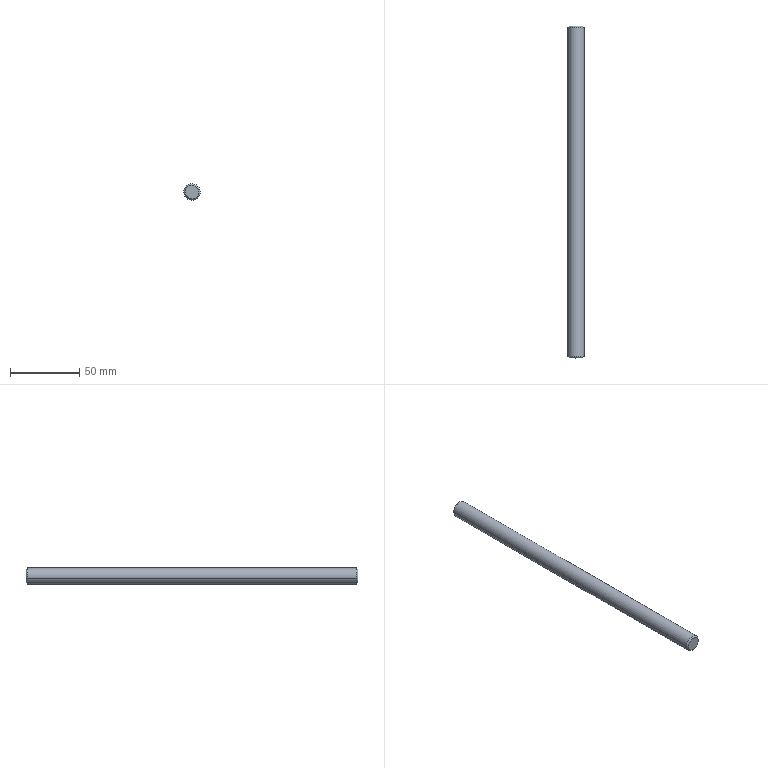Component | SolidWorks | KSD171005A-01-01-21-1 | 1 solid | 8 faces | box 12 x 240 x 12 mm | volume 27108 mm3 | cone 4 | cylinder 2 | plane 2 | commonest cylinder face diameters 12 x2
build123d program:
from build123d import *

# Parameters (mm, degrees)
SKETCH1_R           = 6
BOSS_EXTRUDE1_DEPTH = 240
CHAMFER1_SIZE       = 1


with BuildPart() as part:
    # Sketch1 → Boss-Extrude1 (new body)
    with BuildSketch(Plane.XY):
        Circle(SKETCH1_R)
    extrude(amount=BOSS_EXTRUDE1_DEPTH)

    # Chamfer1
    chamfer1_edges = [part.edges().sort_by_distance(p)[0] for p in [
        (-6, 0, 0),
        (-6, 0, 240),
    ]]
    chamfer(chamfer1_edges, length=CHAMFER1_SIZE)


solid = part.part

# Placed as in the assembly
solid = solid.moved(Location((-7.111, 270.73, 407), (90, 0, 0)))
STEP:
#1=CARTESIAN_POINT('',(-0.09338,1.21,16.086));
#2=VERTEX_POINT('',#1);
#3=CARTESIAN_POINT('',(-0.4666,1.21,15.961));
#4=VERTEX_POINT('',#3);
#5=CARTESIAN_POINT('',(-0.28,1.21,16.024));
#6=DIRECTION('',(0.,-1.,0.));
#7=DIRECTION('',(0.9479,0.,0.3186));
#8=AXIS2_PLACEMENT_3D('',#5,#6,#7);
#9=CIRCLE('',#8,0.1969);
#10=EDGE_CURVE('',#2,#4,#9,.T.);
#11=ORIENTED_EDGE('',*,*,#10,.F.);
#12=CARTESIAN_POINT('',(-0.05607,1.249,16.099));
#13=VERTEX_POINT('',#12);
#14=CARTESIAN_POINT('',(-0.09338,1.21,16.086));
#15=DIRECTION('',(0.6703,0.7071,0.2253));
#16=VECTOR('',#15,39.37);
#17=LINE('',#14,#16);
#18=EDGE_CURVE('',#2,#13,#17,.T.);
#19=ORIENTED_EDGE('',*,*,#18,.T.);
#20=CARTESIAN_POINT('',(-0.5039,1.249,15.948));
#21=VERTEX_POINT('',#20);
#22=CARTESIAN_POINT('',(-0.28,1.249,16.024));
#23=DIRECTION('',(-0.,1.,-0.));
#24=DIRECTION('',(0.9479,0.,0.3186));
#25=AXIS2_PLACEMENT_3D('',#22,#23,#24);
#26=CIRCLE('',#25,0.2362);
#27=EDGE_CURVE('',#21,#13,#26,.T.);
#28=ORIENTED_EDGE('',*,*,#27,.F.);
#29=CARTESIAN_POINT('',(-0.4666,1.21,15.961));
#30=DIRECTION('',(-0.6703,0.7071,-0.2253));
#31=VECTOR('',#30,39.37);
#32=LINE('',#29,#31);
#33=EDGE_CURVE('',#4,#21,#32,.T.);
#34=ORIENTED_EDGE('',*,*,#33,.F.);
#35=EDGE_LOOP('',(#11,#19,#28,#34));
#36=FACE_OUTER_BOUND('',#35,.T.);
#37=CARTESIAN_POINT('',(-0.28,1.21,16.024));
#38=DIRECTION('',(-0.,1.,-0.));
#39=DIRECTION('',(-0.9479,0.,-0.3186));
#40=AXIS2_PLACEMENT_3D('',#37,#38,#39);
#41=CONICAL_SURFACE('',#40,0.1969,0.7854);
#42=ADVANCED_FACE('',(#36),#41,.T.);
#43=CARTESIAN_POINT('',(-0.4666,10.659,15.961));
#44=VERTEX_POINT('',#43);
#45=CARTESIAN_POINT('',(-0.09338,10.659,16.086));
#46=VERTEX_POINT('',#45);
#47=CARTESIAN_POINT('',(-0.28,10.659,16.024));
#48=DIRECTION('',(-0.,1.,-0.));
#49=DIRECTION('',(0.9479,0.,0.3186));
#50=AXIS2_PLACEMENT_3D('',#47,#48,#49);
#51=CIRCLE('',#50,0.1969);
#52=EDGE_CURVE('',#44,#46,#51,.T.);
#53=ORIENTED_EDGE('',*,*,#52,.F.);
#54=CARTESIAN_POINT('',(-0.5039,10.619,15.948));
#55=VERTEX_POINT('',#54);
#56=CARTESIAN_POINT('',(-0.5039,10.619,15.948));
#57=DIRECTION('',(-0.6703,-0.7071,-0.2253));
#58=VECTOR('',#57,39.37);
#59=LINE('',#56,#58);
#60=EDGE_CURVE('',#44,#55,#59,.T.);
#61=ORIENTED_EDGE('',*,*,#60,.T.);
#62=CARTESIAN_POINT('',(-0.05607,10.619,16.099));
#63=VERTEX_POINT('',#62);
#64=CARTESIAN_POINT('',(-0.28,10.619,16.024));
#65=DIRECTION('',(0.,-1.,0.));
#66=DIRECTION('',(0.9479,0.,0.3186));
#67=AXIS2_PLACEMENT_3D('',#64,#65,#66);
#68=CIRCLE('',#67,0.2362);
#69=EDGE_CURVE('',#63,#55,#68,.T.);
#70=ORIENTED_EDGE('',*,*,#69,.F.);
#71=CARTESIAN_POINT('',(-0.05607,10.619,16.099));
#72=DIRECTION('',(0.6703,-0.7071,0.2253));
#73=VECTOR('',#72,39.37);
#74=LINE('',#71,#73);
#75=EDGE_CURVE('',#46,#63,#74,.T.);
#76=ORIENTED_EDGE('',*,*,#75,.F.);
#77=EDGE_LOOP('',(#53,#61,#70,#76));
#78=FACE_OUTER_BOUND('',#77,.T.);
#79=CARTESIAN_POINT('',(-0.28,10.619,16.024));
#80=DIRECTION('',(0.,-1.,0.));
#81=DIRECTION('',(0.9479,0.,0.3186));
#82=AXIS2_PLACEMENT_3D('',#79,#80,#81);
#83=CONICAL_SURFACE('',#82,0.2362,0.7854);
#84=ADVANCED_FACE('',(#78),#83,.T.);
#85=ORIENTED_EDGE('',*,*,#27,.T.);
#86=CARTESIAN_POINT('',(-0.05607,1.21,16.099));
#87=DIRECTION('',(-0.,1.,-0.));
#88=VECTOR('',#87,39.37);
#89=LINE('',#86,#88);
#90=EDGE_CURVE('',#13,#63,#89,.T.);
#91=ORIENTED_EDGE('',*,*,#90,.T.);
#92=ORIENTED_EDGE('',*,*,#69,.T.);
#93=CARTESIAN_POINT('',(-0.5039,1.21,15.948));
#94=DIRECTION('',(-0.,1.,-0.));
#95=VECTOR('',#94,39.37);
#96=LINE('',#93,#95);
#97=EDGE_CURVE('',#21,#55,#96,.T.);
#98=ORIENTED_EDGE('',*,*,#97,.F.);
#99=EDGE_LOOP('',(#85,#91,#92,#98));
#100=FACE_OUTER_BOUND('',#99,.T.);
#101=CARTESIAN_POINT('',(-0.28,1.21,16.024));
#102=DIRECTION('',(-0.,1.,-0.));
#103=DIRECTION('',(-0.9479,0.,-0.3186));
#104=AXIS2_PLACEMENT_3D('',#101,#102,#103);
#105=CYLINDRICAL_SURFACE('',#104,0.2362);
#106=ADVANCED_FACE('',(#100),#105,.T.);
#107=ORIENTED_EDGE('',*,*,#90,.F.);
#108=CARTESIAN_POINT('',(-0.28,1.249,16.024));
#109=DIRECTION('',(-0.,1.,-0.));
#110=DIRECTION('',(0.9479,0.,0.3186));
#111=AXIS2_PLACEMENT_3D('',#108,#109,#110);
#112=CIRCLE('',#111,0.2362);
#113=EDGE_CURVE('',#13,#21,#112,.T.);
#114=ORIENTED_EDGE('',*,*,#113,.T.);
#115=ORIENTED_EDGE('',*,*,#97,.T.);
#116=CARTESIAN_POINT('',(-0.28,10.619,16.024));
#117=DIRECTION('',(0.,-1.,0.));
#118=DIRECTION('',(0.9479,0.,0.3186));
#119=AXIS2_PLACEMENT_3D('',#116,#117,#118);
#120=CIRCLE('',#119,0.2362);
#121=EDGE_CURVE('',#55,#63,#120,.T.);
#122=ORIENTED_EDGE('',*,*,#121,.T.);
#123=EDGE_LOOP('',(#107,#114,#115,#122));
#124=FACE_OUTER_BOUND('',#123,.T.);
#125=CARTESIAN_POINT('',(-0.28,1.21,16.024));
#126=DIRECTION('',(-0.,1.,-0.));
#127=DIRECTION('',(-0.9479,0.,-0.3186));
#128=AXIS2_PLACEMENT_3D('',#125,#126,#127);
#129=CYLINDRICAL_SURFACE('',#128,0.2362);
#130=ADVANCED_FACE('',(#124),#129,.T.);
#131=CARTESIAN_POINT('',(-0.28,1.21,16.024));
#132=DIRECTION('',(0.,-1.,0.));
#133=DIRECTION('',(0.9479,0.,0.3186));
#134=AXIS2_PLACEMENT_3D('',#131,#132,#133);
#135=CIRCLE('',#134,0.1969);
#136=EDGE_CURVE('',#4,#2,#135,.T.);
#137=ORIENTED_EDGE('',*,*,#136,.T.);
#138=ORIENTED_EDGE('',*,*,#10,.T.);
#139=EDGE_LOOP('',(#137,#138));
#140=FACE_OUTER_BOUND('',#139,.T.);
#141=CARTESIAN_POINT('',(-0.28,1.21,16.024));
#142=DIRECTION('',(0.,-1.,0.));
#143=DIRECTION('',(0.9479,0.,0.3186));
#144=AXIS2_PLACEMENT_3D('',#141,#142,#143);
#145=PLANE('',#144);
#146=ADVANCED_FACE('',(#140),#145,.T.);
#147=CARTESIAN_POINT('',(-0.28,10.659,16.024));
#148=DIRECTION('',(-0.,1.,-0.));
#149=DIRECTION('',(0.9479,0.,0.3186));
#150=AXIS2_PLACEMENT_3D('',#147,#148,#149);
#151=CIRCLE('',#150,0.1969);
#152=EDGE_CURVE('',#46,#44,#151,.T.);
#153=ORIENTED_EDGE('',*,*,#152,.T.);
#154=ORIENTED_EDGE('',*,*,#52,.T.);
#155=EDGE_LOOP('',(#153,#154));
#156=FACE_OUTER_BOUND('',#155,.T.);
#157=CARTESIAN_POINT('',(-0.28,10.659,16.024));
#158=DIRECTION('',(0.,-1.,0.));
#159=DIRECTION('',(0.9479,0.,0.3186));
#160=AXIS2_PLACEMENT_3D('',#157,#158,#159);
#161=PLANE('',#160);
#162=ADVANCED_FACE('',(#156),#161,.F.);
#163=ORIENTED_EDGE('',*,*,#60,.F.);
#164=ORIENTED_EDGE('',*,*,#152,.F.);
#165=ORIENTED_EDGE('',*,*,#75,.T.);
#166=ORIENTED_EDGE('',*,*,#121,.F.);
#167=EDGE_LOOP('',(#163,#164,#165,#166));
#168=FACE_OUTER_BOUND('',#167,.T.);
#169=CARTESIAN_POINT('',(-0.28,10.619,16.024));
#170=DIRECTION('',(0.,-1.,0.));
#171=DIRECTION('',(0.9479,0.,0.3186));
#172=AXIS2_PLACEMENT_3D('',#169,#170,#171);
#173=CONICAL_SURFACE('',#172,0.2362,0.7854);
#174=ADVANCED_FACE('',(#168),#173,.T.);
#175=ORIENTED_EDGE('',*,*,#18,.F.);
#176=ORIENTED_EDGE('',*,*,#136,.F.);
#177=ORIENTED_EDGE('',*,*,#33,.T.);
#178=ORIENTED_EDGE('',*,*,#113,.F.);
#179=EDGE_LOOP('',(#175,#176,#177,#178));
#180=FACE_OUTER_BOUND('',#179,.T.);
#181=CARTESIAN_POINT('',(-0.28,1.21,16.024));
#182=DIRECTION('',(-0.,1.,-0.));
#183=DIRECTION('',(-0.9479,0.,-0.3186));
#184=AXIS2_PLACEMENT_3D('',#181,#182,#183);
#185=CONICAL_SURFACE('',#184,0.1969,0.7854);
#186=ADVANCED_FACE('',(#180),#185,.T.);
#187=CLOSED_SHELL('',(#42,#84,#106,#130,#146,#162,#174,#186));
#188=MANIFOLD_SOLID_BREP('',#187);
#189=CARTESIAN_POINT('',(0.,0.,0.));
#190=DIRECTION('',(0.,0.,1.));
#191=DIRECTION('',(1.,0.,0.));
#192=AXIS2_PLACEMENT_3D('',#189,#190,#191);
#193=(LENGTH_UNIT()NAMED_UNIT(*)SI_UNIT($,.METRE.));
#194=LENGTH_MEASURE_WITH_UNIT(LENGTH_MEASURE(0.0254),#193);
#195=DIMENSIONAL_EXPONENTS(1.,0.,0.,0.,0.,0.,0.);
#196=(CONVERSION_BASED_UNIT('',#194)LENGTH_UNIT()NAMED_UNIT(#195));
#197=UNCERTAINTY_MEASURE_WITH_UNIT(LENGTH_MEASURE(0.00001),#196,'','');
#198=(NAMED_UNIT(*)PLANE_ANGLE_UNIT()SI_UNIT($,.RADIAN.));
#199=(NAMED_UNIT(*)SI_UNIT($,.STERADIAN.)SOLID_ANGLE_UNIT());
#200=(GEOMETRIC_REPRESENTATION_CONTEXT(3)GLOBAL_UNCERTAINTY_ASSIGNED_CONTEXT((#197))GLOBAL_UNIT_ASSIGNED_CONTEXT((#196,#198,#199))REPRESENTATION_CONTEXT('',''));
#201=ADVANCED_BREP_SHAPE_REPRESENTATION('',(#188,#192),#200);
#202=COLOUR_RGB('',0.7922,0.8196,0.9333);
#203=FILL_AREA_STYLE_COLOUR('',#202);
#204=FILL_AREA_STYLE('',(#203));
#205=SURFACE_STYLE_FILL_AREA(#204);
#206=SURFACE_SIDE_STYLE('',(#205));
#207=SURFACE_STYLE_USAGE(.BOTH.,#206);
#208=PRESENTATION_STYLE_ASSIGNMENT((#207));
#209=STYLED_ITEM('',(#208),#188);
#210=PRESENTATION_LAYER_ASSIGNMENT('','',(#209));
#211=(LENGTH_UNIT()NAMED_UNIT(*)SI_UNIT($,.METRE.));
#212=LENGTH_MEASURE_WITH_UNIT(LENGTH_MEASURE(0.0254),#211);
#213=DIMENSIONAL_EXPONENTS(1.,0.,0.,0.,0.,0.,0.);
#214=(CONVERSION_BASED_UNIT('',#212)LENGTH_UNIT()NAMED_UNIT(#213));
#215=UNCERTAINTY_MEASURE_WITH_UNIT(LENGTH_MEASURE(0.00001),#214,'','');
#216=(NAMED_UNIT(*)PLANE_ANGLE_UNIT()SI_UNIT($,.RADIAN.));
#217=(NAMED_UNIT(*)SI_UNIT($,.STERADIAN.)SOLID_ANGLE_UNIT());
#218=(GEOMETRIC_REPRESENTATION_CONTEXT(3)GLOBAL_UNCERTAINTY_ASSIGNED_CONTEXT((#215))GLOBAL_UNIT_ASSIGNED_CONTEXT((#214,#216,#217))REPRESENTATION_CONTEXT('',''));
#219=MECHANICAL_DESIGN_GEOMETRIC_PRESENTATION_REPRESENTATION('',(#209),#218);